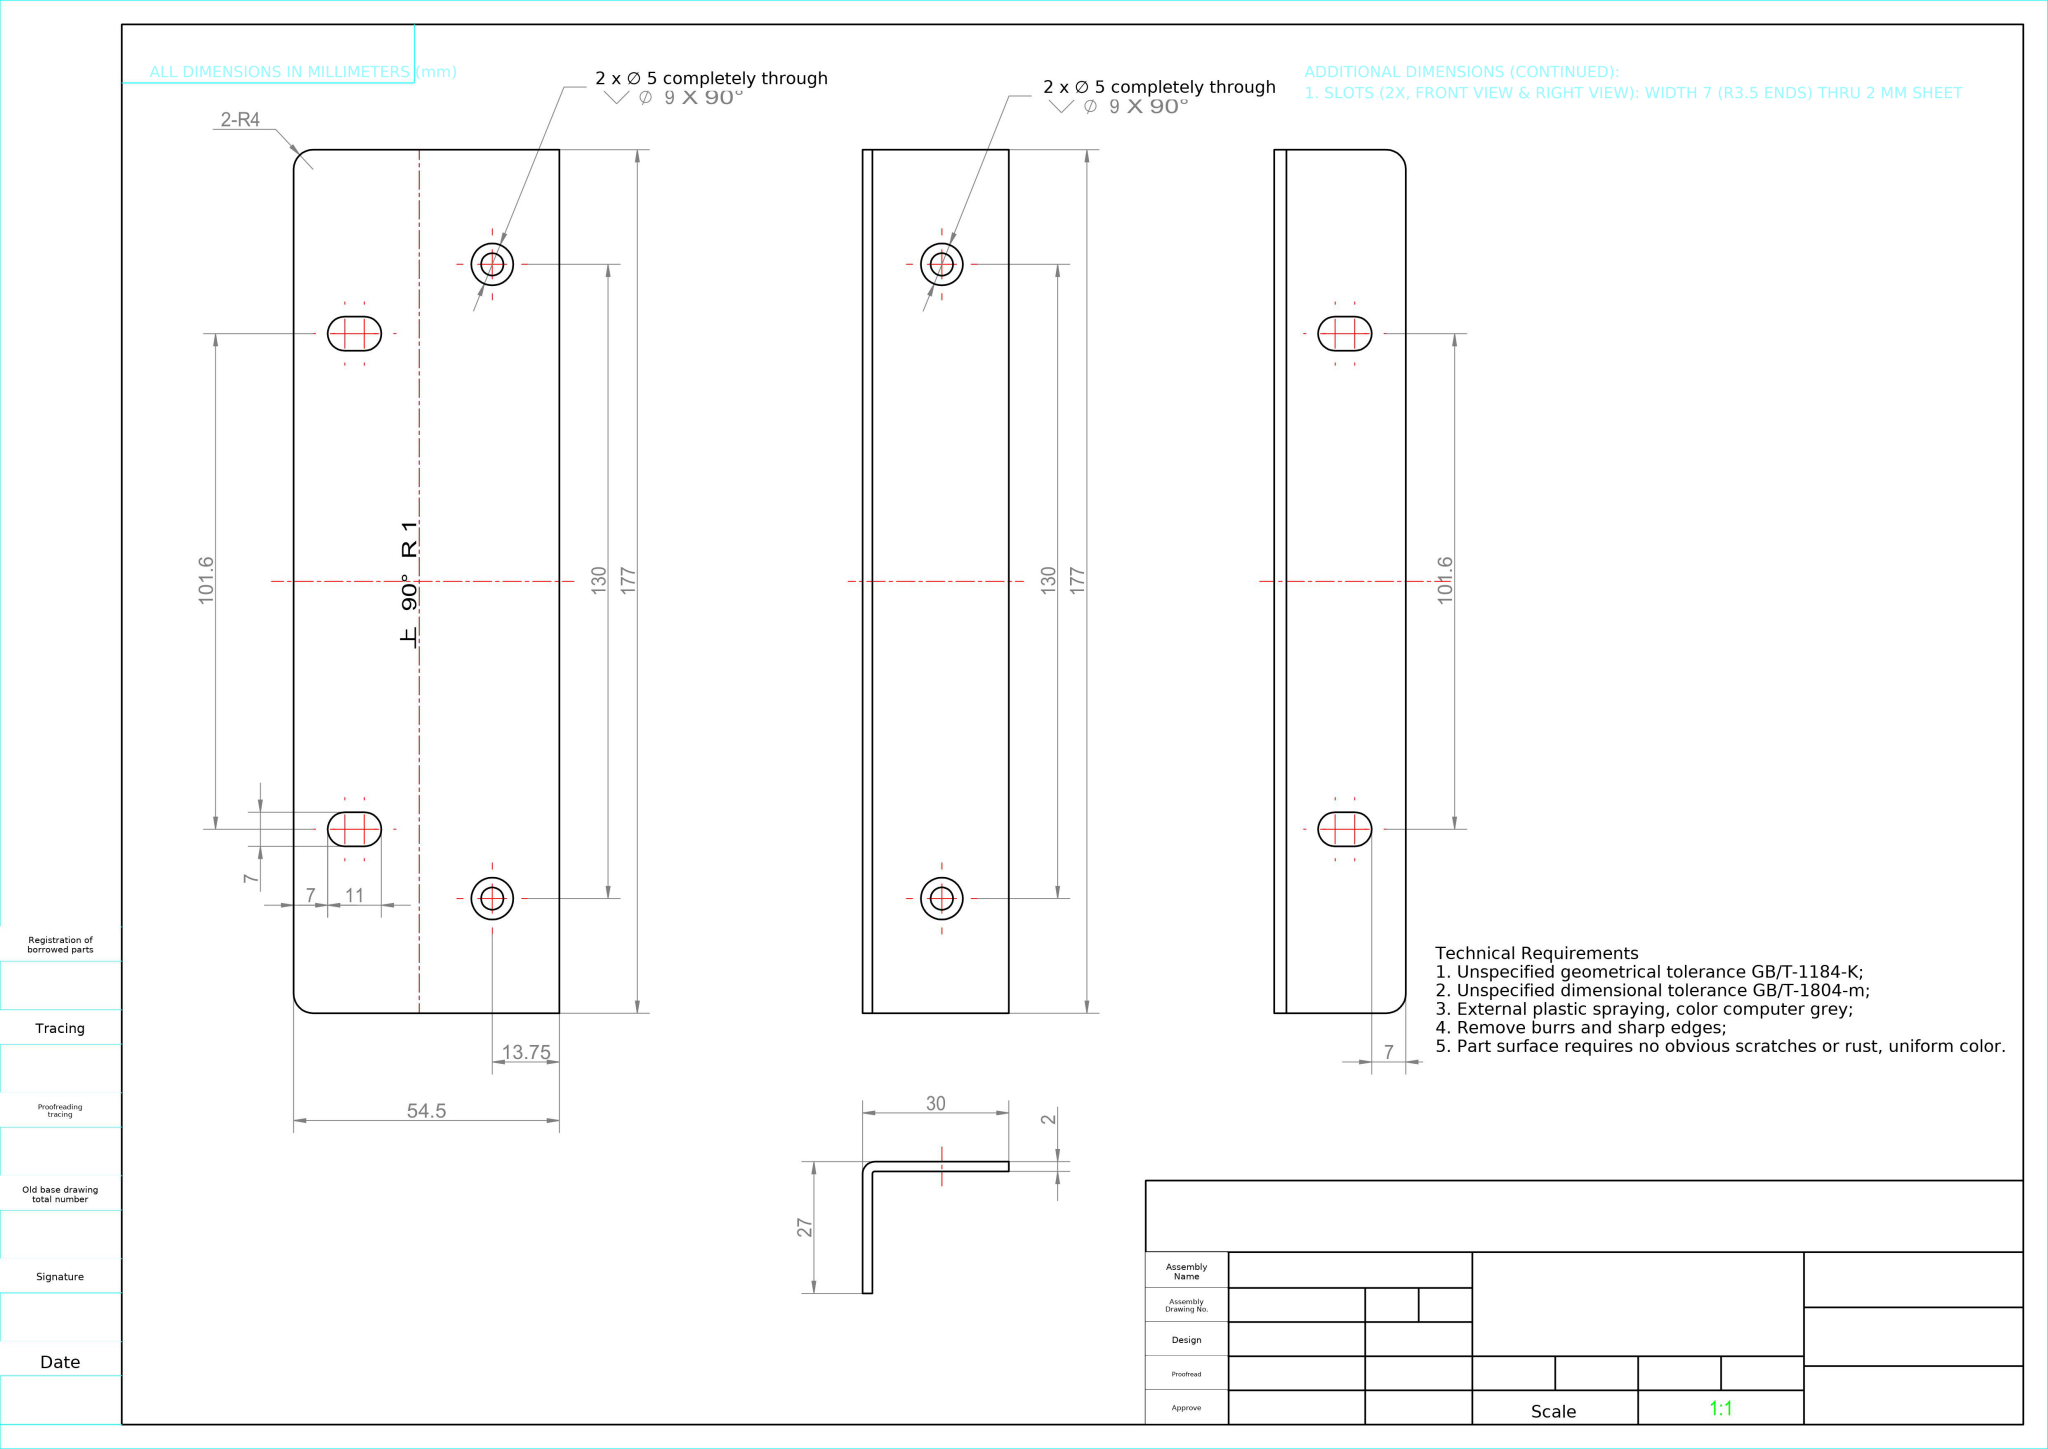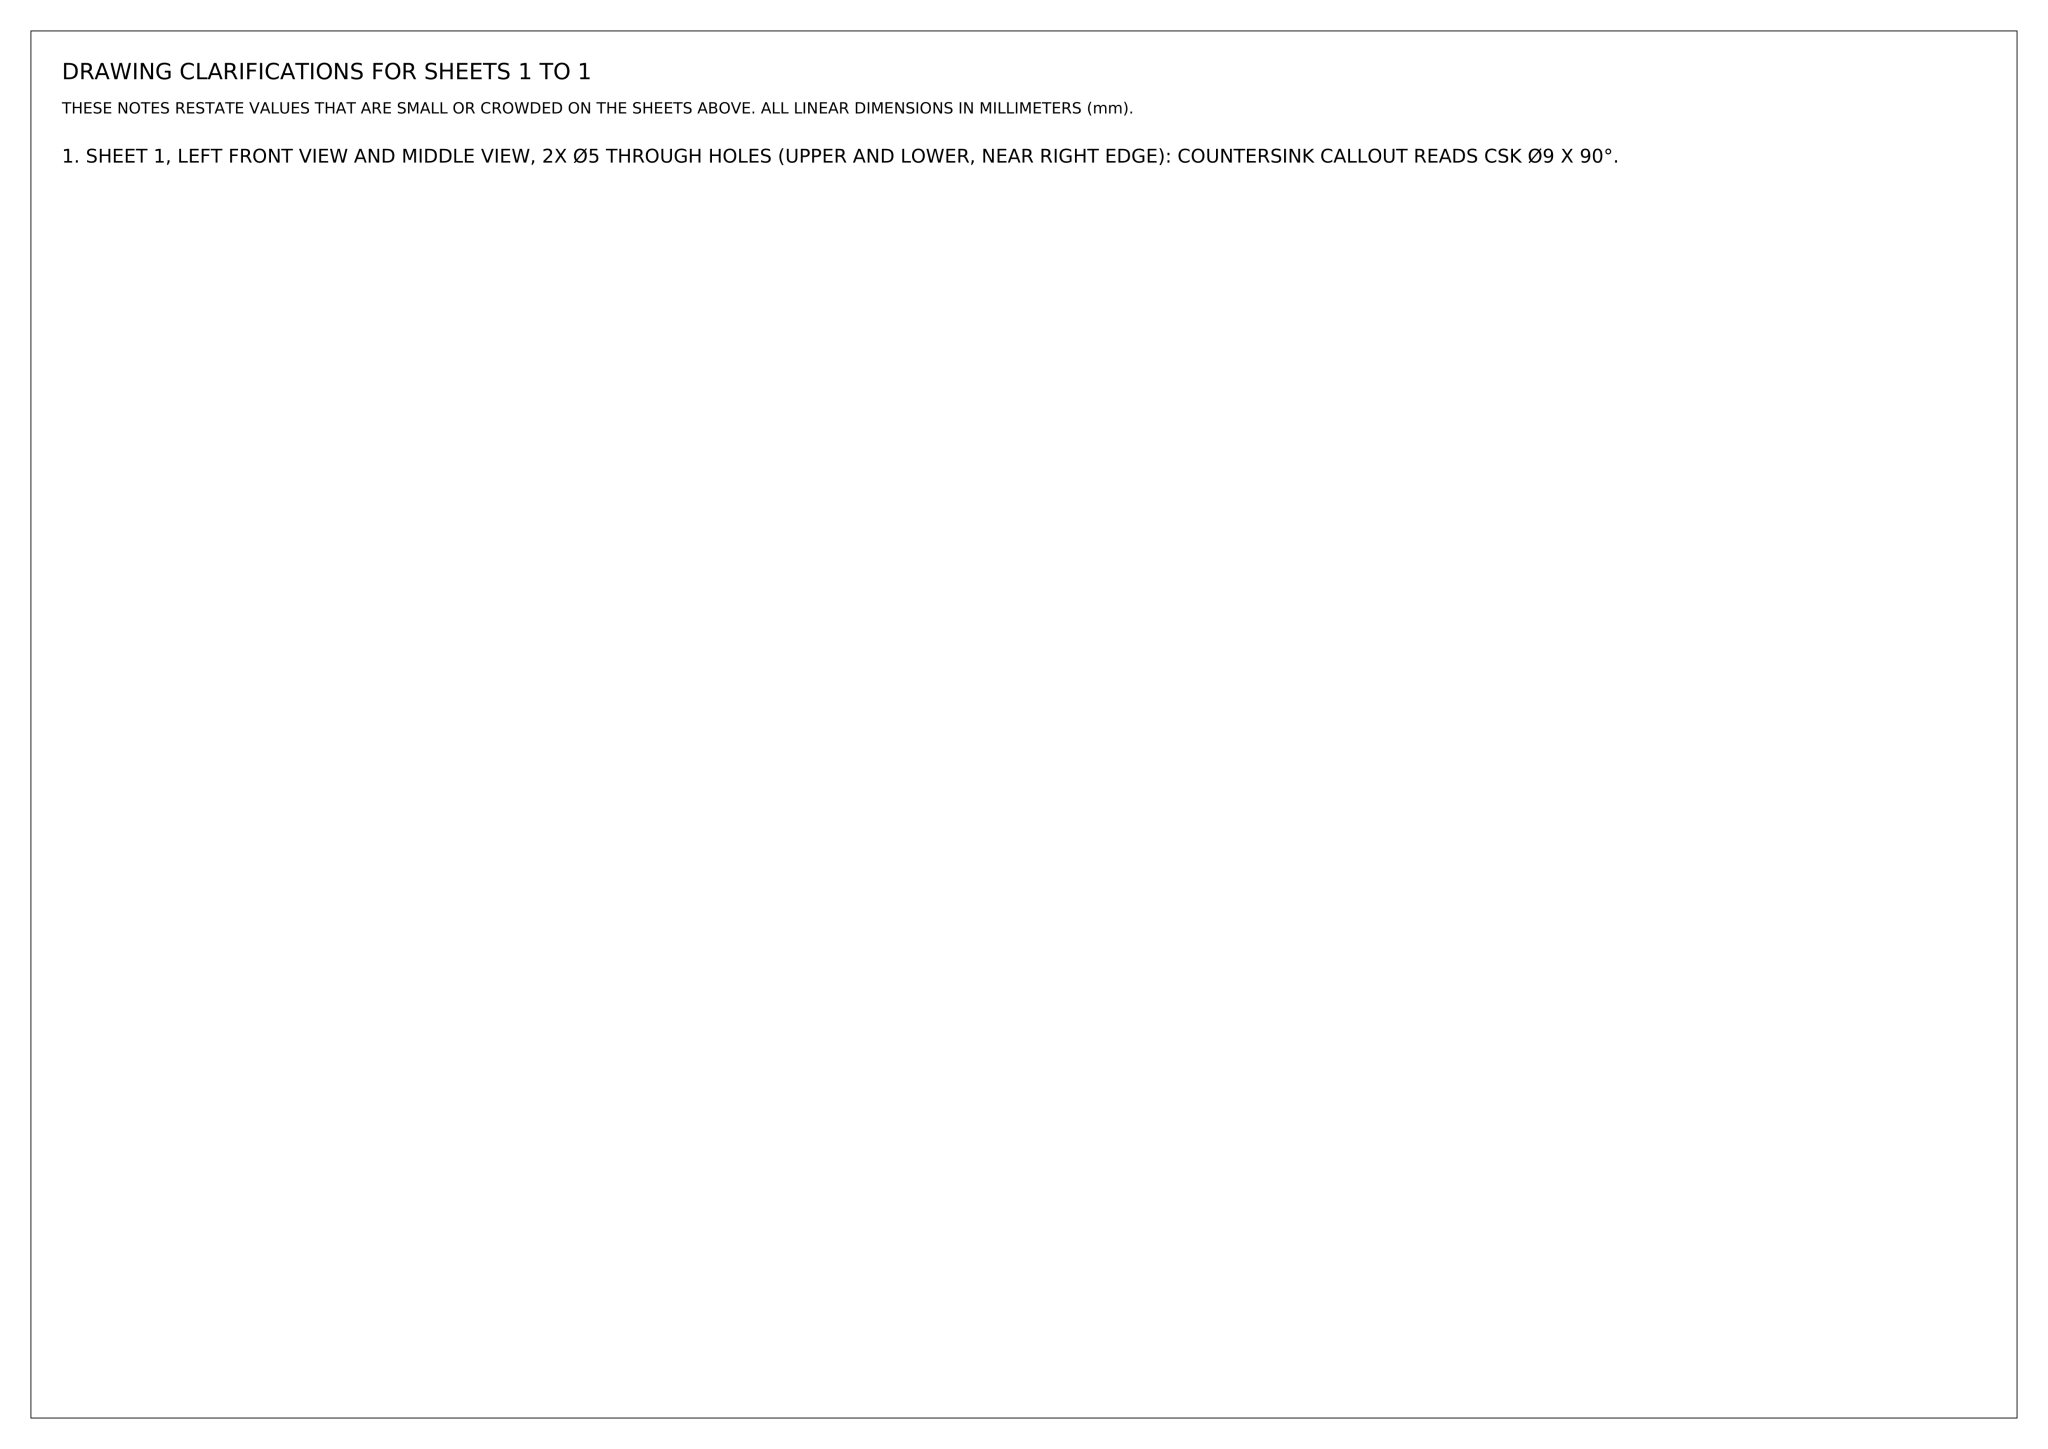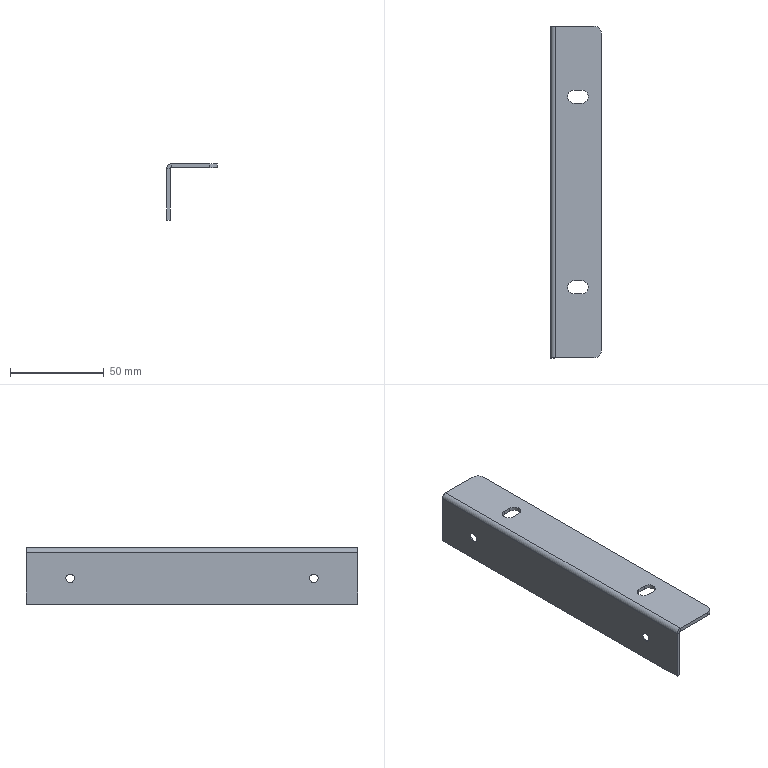Part | NX | mm | 1 solid | 30 faces | box 27 x 177 x 30 mm | volume 18821 mm3 | plane 16 | cylinder 10 | cone 4 | commonest cylinder face diameters 7 x6 8 x2 1 x1 5 x1